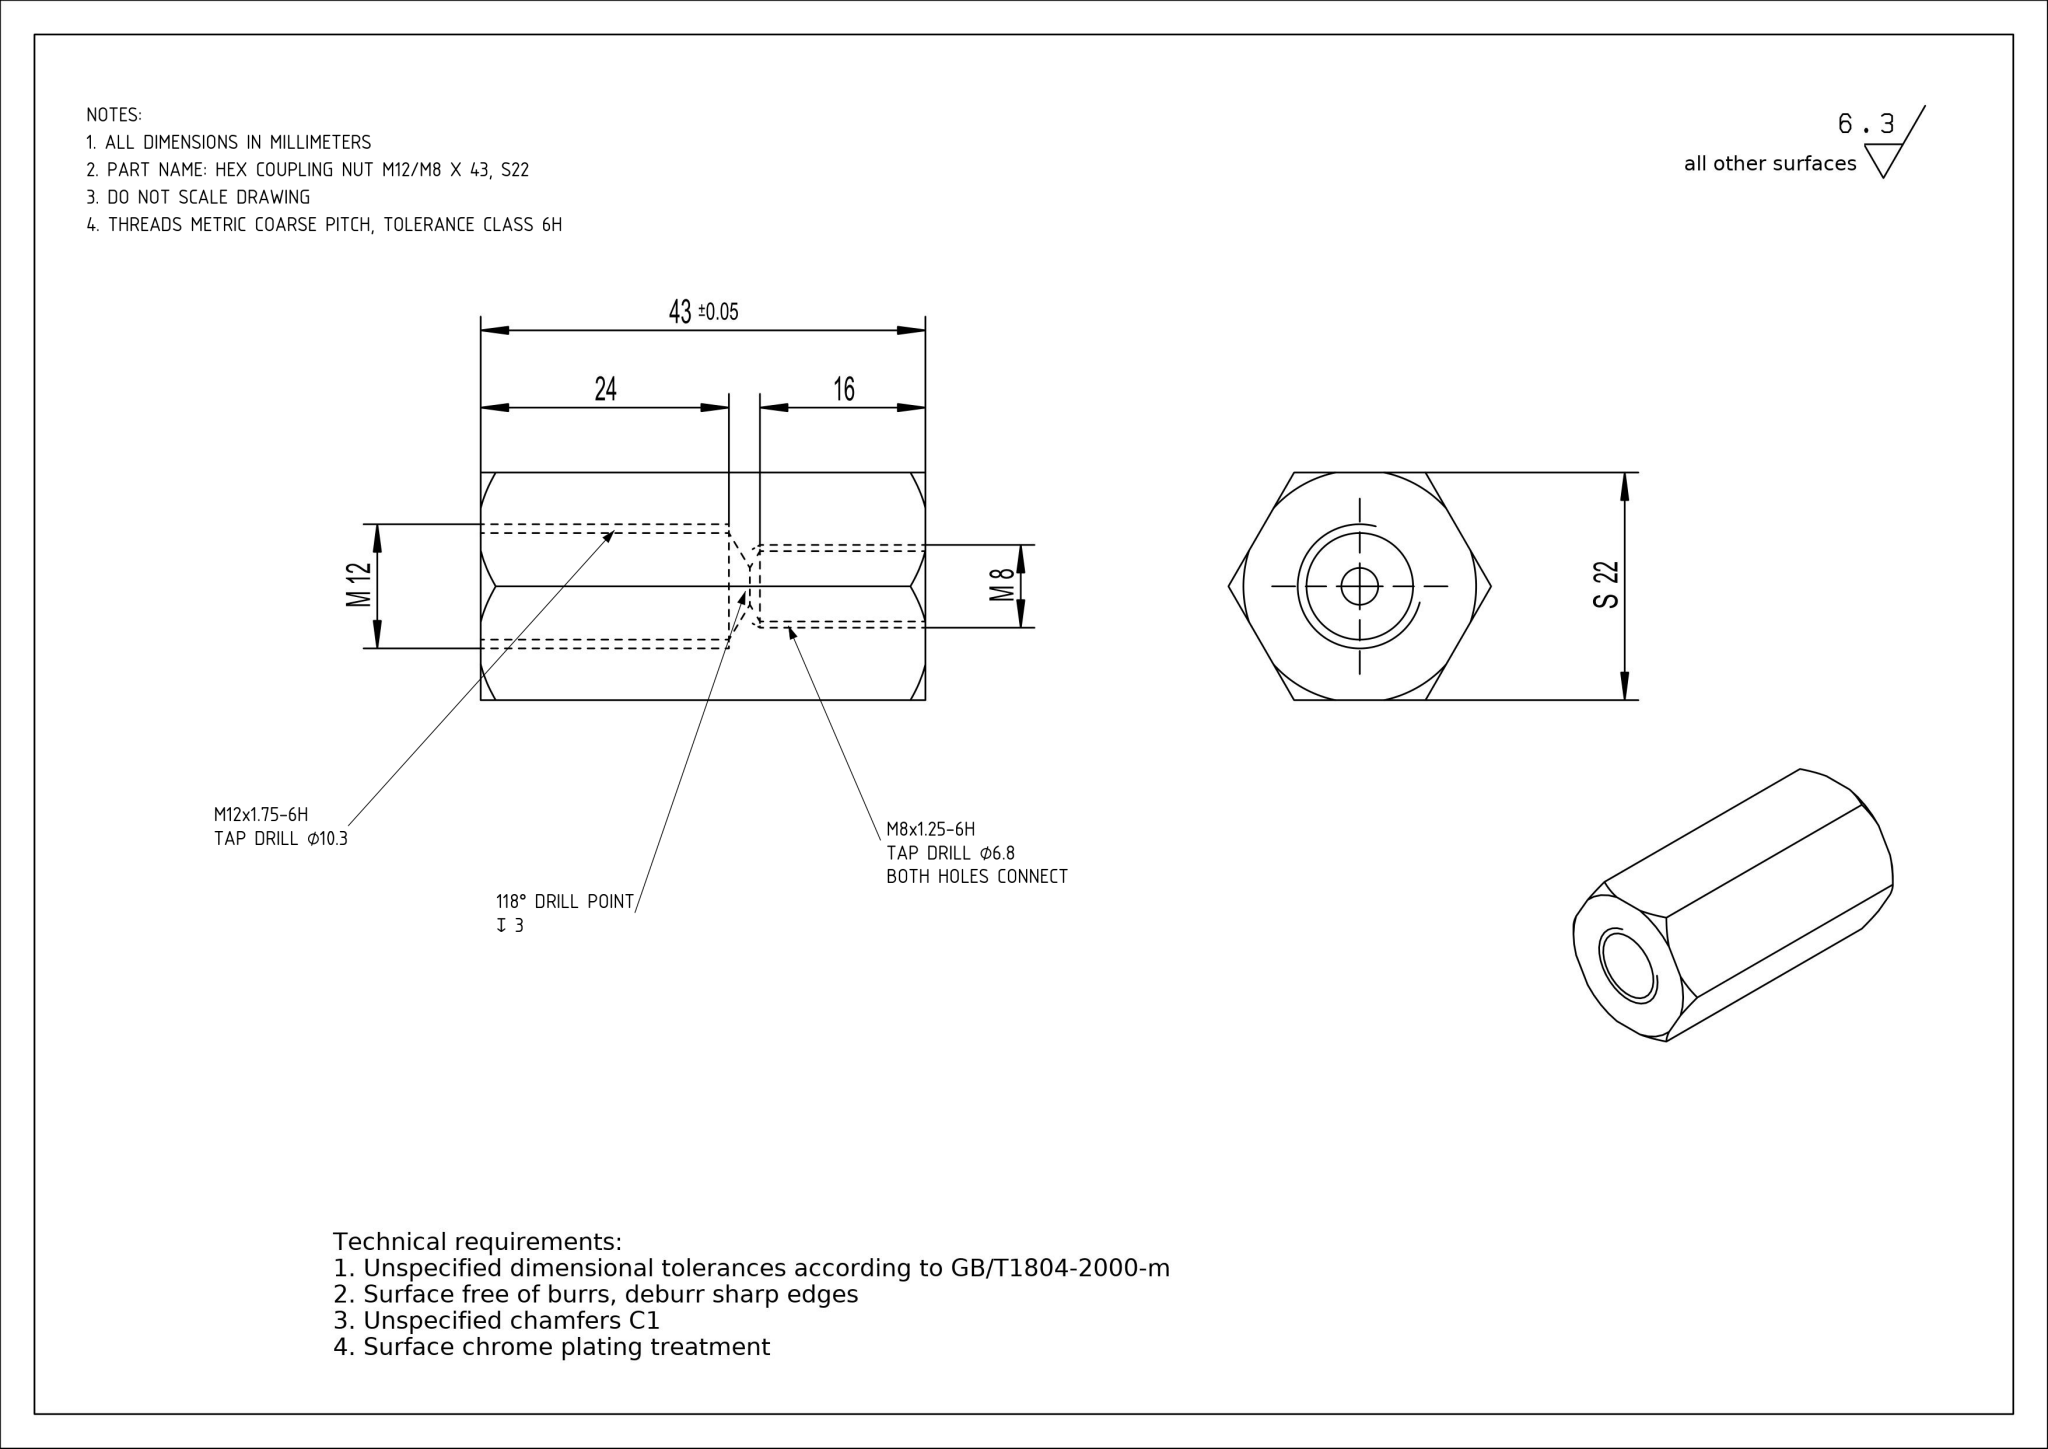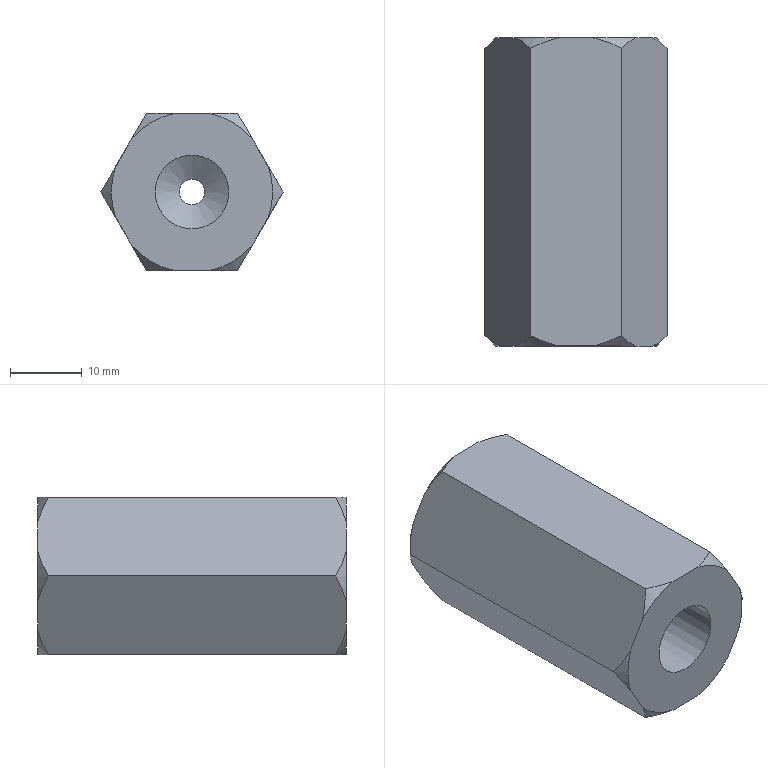Part | NX | mm | 1 solid | 24 faces | box 25.4 x 43 x 22 mm | volume 15315 mm3 | cone 14 | plane 8 | cylinder 2 | commonest cylinder face diameters 6.8 x1 10.3 x1
STEP:
#1=CARTESIAN_POINT('',(0.,0.,0.));
#2=DIRECTION('',(0.,0.,1.));
#3=DIRECTION('',(1.,0.,0.));
#4=AXIS2_PLACEMENT_3D('',#1,#2,#3);
#5=(LENGTH_UNIT()NAMED_UNIT(*)SI_UNIT(.MILLI.,.METRE.));
#6=UNCERTAINTY_MEASURE_WITH_UNIT(LENGTH_MEASURE(0.0508),#5,'','');
#7=(NAMED_UNIT(*)PLANE_ANGLE_UNIT()SI_UNIT($,.RADIAN.));
#8=PLANE_ANGLE_MEASURE_WITH_UNIT(PLANE_ANGLE_MEASURE(0.01745),#7);
#9=DIMENSIONAL_EXPONENTS(0.,0.,0.,0.,0.,0.,0.);
#10=(CONVERSION_BASED_UNIT('',#8)NAMED_UNIT(#9)PLANE_ANGLE_UNIT());
#11=(NAMED_UNIT(*)SI_UNIT($,.STERADIAN.)SOLID_ANGLE_UNIT());
#12=(GEOMETRIC_REPRESENTATION_CONTEXT(3)GLOBAL_UNCERTAINTY_ASSIGNED_CONTEXT((#6))GLOBAL_UNIT_ASSIGNED_CONTEXT((#5,#10,#11))REPRESENTATION_CONTEXT('',''));
#13=SHAPE_REPRESENTATION('',(#4),#12);
#14=CARTESIAN_POINT('',(0.,0.,5.15));
#15=VERTEX_POINT('',#14);
#16=CARTESIAN_POINT('',(0.,0.,0.));
#17=DIRECTION('',(0.,1.,0.));
#18=DIRECTION('',(0.,0.,1.));
#19=AXIS2_PLACEMENT_3D('',#16,#17,#18);
#20=CIRCLE('',#19,5.15);
#21=EDGE_CURVE('',#15,#15,#20,.T.);
#22=ORIENTED_EDGE('',*,*,#21,.T.);
#23=EDGE_LOOP('',(#22));
#24=FACE_BOUND('',#23,.T.);
#25=CARTESIAN_POINT('',(-8.347,0.,7.543));
#26=VERTEX_POINT('',#25);
#27=CARTESIAN_POINT('',(-2.358,0.,11.));
#28=VERTEX_POINT('',#27);
#29=CARTESIAN_POINT('',(0.,0.,-0.));
#30=DIRECTION('',(0.,1.,0.));
#31=DIRECTION('',(-1.,0.,-0.));
#32=AXIS2_PLACEMENT_3D('',#29,#30,#31);
#33=CIRCLE('',#32,11.25);
#34=EDGE_CURVE('',#26,#28,#33,.T.);
#35=ORIENTED_EDGE('',*,*,#34,.F.);
#36=CARTESIAN_POINT('',(-10.706,0.,3.457));
#37=VERTEX_POINT('',#36);
#38=CARTESIAN_POINT('',(-6.351,0.,11.));
#39=DIRECTION('',(-0.5,0.,-0.866));
#40=VECTOR('',#39,1.);
#41=LINE('',#38,#40);
#42=EDGE_CURVE('',#26,#37,#41,.T.);
#43=ORIENTED_EDGE('',*,*,#42,.T.);
#44=CARTESIAN_POINT('',(-10.706,0.,-3.457));
#45=VERTEX_POINT('',#44);
#46=CARTESIAN_POINT('',(0.,0.,-0.));
#47=DIRECTION('',(0.,1.,0.));
#48=DIRECTION('',(-1.,0.,-0.));
#49=AXIS2_PLACEMENT_3D('',#46,#47,#48);
#50=CIRCLE('',#49,11.25);
#51=EDGE_CURVE('',#45,#37,#50,.T.);
#52=ORIENTED_EDGE('',*,*,#51,.F.);
#53=CARTESIAN_POINT('',(-8.347,0.,-7.543));
#54=VERTEX_POINT('',#53);
#55=CARTESIAN_POINT('',(-12.702,0.,0.));
#56=DIRECTION('',(0.5,0.,-0.866));
#57=VECTOR('',#56,1.);
#58=LINE('',#55,#57);
#59=EDGE_CURVE('',#45,#54,#58,.T.);
#60=ORIENTED_EDGE('',*,*,#59,.T.);
#61=CARTESIAN_POINT('',(-2.358,0.,-11.));
#62=VERTEX_POINT('',#61);
#63=CARTESIAN_POINT('',(0.,0.,-0.));
#64=DIRECTION('',(0.,1.,0.));
#65=DIRECTION('',(-1.,0.,-0.));
#66=AXIS2_PLACEMENT_3D('',#63,#64,#65);
#67=CIRCLE('',#66,11.25);
#68=EDGE_CURVE('',#62,#54,#67,.T.);
#69=ORIENTED_EDGE('',*,*,#68,.F.);
#70=CARTESIAN_POINT('',(2.358,0.,-11.));
#71=VERTEX_POINT('',#70);
#72=CARTESIAN_POINT('',(-6.351,0.,-11.));
#73=DIRECTION('',(1.,0.,-0.));
#74=VECTOR('',#73,1.);
#75=LINE('',#72,#74);
#76=EDGE_CURVE('',#62,#71,#75,.T.);
#77=ORIENTED_EDGE('',*,*,#76,.T.);
#78=CARTESIAN_POINT('',(8.347,0.,-7.543));
#79=VERTEX_POINT('',#78);
#80=CARTESIAN_POINT('',(0.,0.,-0.));
#81=DIRECTION('',(0.,1.,0.));
#82=DIRECTION('',(-1.,0.,-0.));
#83=AXIS2_PLACEMENT_3D('',#80,#81,#82);
#84=CIRCLE('',#83,11.25);
#85=EDGE_CURVE('',#79,#71,#84,.T.);
#86=ORIENTED_EDGE('',*,*,#85,.F.);
#87=CARTESIAN_POINT('',(10.706,0.,-3.457));
#88=VERTEX_POINT('',#87);
#89=CARTESIAN_POINT('',(6.351,0.,-11.));
#90=DIRECTION('',(0.5,0.,0.866));
#91=VECTOR('',#90,1.);
#92=LINE('',#89,#91);
#93=EDGE_CURVE('',#79,#88,#92,.T.);
#94=ORIENTED_EDGE('',*,*,#93,.T.);
#95=CARTESIAN_POINT('',(10.706,0.,3.457));
#96=VERTEX_POINT('',#95);
#97=CARTESIAN_POINT('',(0.,0.,-0.));
#98=DIRECTION('',(0.,1.,0.));
#99=DIRECTION('',(-1.,0.,-0.));
#100=AXIS2_PLACEMENT_3D('',#97,#98,#99);
#101=CIRCLE('',#100,11.25);
#102=EDGE_CURVE('',#96,#88,#101,.T.);
#103=ORIENTED_EDGE('',*,*,#102,.F.);
#104=CARTESIAN_POINT('',(8.347,0.,7.543));
#105=VERTEX_POINT('',#104);
#106=CARTESIAN_POINT('',(12.702,0.,-0.));
#107=DIRECTION('',(-0.5,0.,0.866));
#108=VECTOR('',#107,1.);
#109=LINE('',#106,#108);
#110=EDGE_CURVE('',#96,#105,#109,.T.);
#111=ORIENTED_EDGE('',*,*,#110,.T.);
#112=CARTESIAN_POINT('',(2.358,0.,11.));
#113=VERTEX_POINT('',#112);
#114=CARTESIAN_POINT('',(0.,0.,-0.));
#115=DIRECTION('',(0.,1.,0.));
#116=DIRECTION('',(-1.,0.,-0.));
#117=AXIS2_PLACEMENT_3D('',#114,#115,#116);
#118=CIRCLE('',#117,11.25);
#119=EDGE_CURVE('',#113,#105,#118,.T.);
#120=ORIENTED_EDGE('',*,*,#119,.F.);
#121=CARTESIAN_POINT('',(6.351,0.,11.));
#122=DIRECTION('',(-1.,0.,0.));
#123=VECTOR('',#122,1.);
#124=LINE('',#121,#123);
#125=EDGE_CURVE('',#113,#28,#124,.T.);
#126=ORIENTED_EDGE('',*,*,#125,.T.);
#127=EDGE_LOOP('',(#35,#43,#52,#60,#69,#77,#86,#94,#103,#111,#120,#126));
#128=FACE_BOUND('',#127,.T.);
#129=CARTESIAN_POINT('',(0.,0.,0.));
#130=DIRECTION('',(0.,-1.,0.));
#131=DIRECTION('',(0.,0.,-1.));
#132=AXIS2_PLACEMENT_3D('',#129,#130,#131);
#133=PLANE('',#132);
#134=ADVANCED_FACE('',(#24,#128),#133,.T.);
#135=CARTESIAN_POINT('',(-6.351,1.452,-11.));
#136=VERTEX_POINT('',#135);
#137=CARTESIAN_POINT('',(-6.351,41.548,-11.));
#138=VERTEX_POINT('',#137);
#139=CARTESIAN_POINT('',(-6.351,0.,-11.));
#140=DIRECTION('',(0.,1.,0.));
#141=VECTOR('',#140,1.);
#142=LINE('',#139,#141);
#143=EDGE_CURVE('',#136,#138,#142,.T.);
#144=ORIENTED_EDGE('',*,*,#143,.F.);
#145=CARTESIAN_POINT('',(-6.351,1.452,-11.));
#146=CARTESIAN_POINT('',(-6.985,0.8177,-9.902));
#147=CARTESIAN_POINT('',(-7.653,0.2911,-8.745));
#148=CARTESIAN_POINT('',(-8.347,-0.,-7.543));
#149=B_SPLINE_CURVE_WITH_KNOTS('',3,(#145,#146,#147,#148),.UNSPECIFIED.,.F.,.F.,(4,4),(0.,1.),.UNSPECIFIED.);
#150=EDGE_CURVE('',#136,#54,#149,.T.);
#151=ORIENTED_EDGE('',*,*,#150,.T.);
#152=ORIENTED_EDGE('',*,*,#59,.F.);
#153=CARTESIAN_POINT('',(-12.702,1.452,0.));
#154=VERTEX_POINT('',#153);
#155=CARTESIAN_POINT('',(-10.706,-0.,-3.457));
#156=CARTESIAN_POINT('',(-11.399,0.2907,-2.257));
#157=CARTESIAN_POINT('',(-12.071,0.8206,-1.093));
#158=CARTESIAN_POINT('',(-12.702,1.452,0.));
#159=B_SPLINE_CURVE_WITH_KNOTS('',3,(#155,#156,#157,#158),.UNSPECIFIED.,.F.,.F.,(4,4),(0.,1.),.UNSPECIFIED.);
#160=EDGE_CURVE('',#45,#154,#159,.T.);
#161=ORIENTED_EDGE('',*,*,#160,.T.);
#162=CARTESIAN_POINT('',(-12.702,41.548,0.));
#163=VERTEX_POINT('',#162);
#164=CARTESIAN_POINT('',(-12.702,0.,0.));
#165=DIRECTION('',(0.,1.,0.));
#166=VECTOR('',#165,1.);
#167=LINE('',#164,#166);
#168=EDGE_CURVE('',#154,#163,#167,.T.);
#169=ORIENTED_EDGE('',*,*,#168,.T.);
#170=CARTESIAN_POINT('',(-10.706,43.,-3.457));
#171=VERTEX_POINT('',#170);
#172=CARTESIAN_POINT('',(-10.706,43.,-3.457));
#173=CARTESIAN_POINT('',(-11.399,42.709,-2.257));
#174=CARTESIAN_POINT('',(-12.071,42.179,-1.093));
#175=CARTESIAN_POINT('',(-12.702,41.548,0.));
#176=B_SPLINE_CURVE_WITH_KNOTS('',3,(#172,#173,#174,#175),.UNSPECIFIED.,.F.,.F.,(4,4),(0.,1.),.UNSPECIFIED.);
#177=EDGE_CURVE('',#171,#163,#176,.T.);
#178=ORIENTED_EDGE('',*,*,#177,.F.);
#179=CARTESIAN_POINT('',(-8.347,43.,-7.543));
#180=VERTEX_POINT('',#179);
#181=CARTESIAN_POINT('',(-12.702,43.,0.));
#182=DIRECTION('',(0.5,0.,-0.866));
#183=VECTOR('',#182,1.);
#184=LINE('',#181,#183);
#185=EDGE_CURVE('',#171,#180,#184,.T.);
#186=ORIENTED_EDGE('',*,*,#185,.T.);
#187=CARTESIAN_POINT('',(-6.351,41.548,-11.));
#188=CARTESIAN_POINT('',(-6.985,42.182,-9.902));
#189=CARTESIAN_POINT('',(-7.653,42.709,-8.745));
#190=CARTESIAN_POINT('',(-8.347,43.,-7.543));
#191=B_SPLINE_CURVE_WITH_KNOTS('',3,(#187,#188,#189,#190),.UNSPECIFIED.,.F.,.F.,(4,4),(0.,1.),.UNSPECIFIED.);
#192=EDGE_CURVE('',#138,#180,#191,.T.);
#193=ORIENTED_EDGE('',*,*,#192,.F.);
#194=EDGE_LOOP('',(#144,#151,#152,#161,#169,#178,#186,#193));
#195=FACE_OUTER_BOUND('',#194,.T.);
#196=CARTESIAN_POINT('',(-12.702,0.,0.));
#197=DIRECTION('',(0.866,0.,0.5));
#198=DIRECTION('',(0.5,0.,-0.866));
#199=AXIS2_PLACEMENT_3D('',#196,#197,#198);
#200=PLANE('',#199);
#201=ADVANCED_FACE('',(#195),#200,.F.);
#202=CARTESIAN_POINT('',(6.351,1.452,-11.));
#203=VERTEX_POINT('',#202);
#204=CARTESIAN_POINT('',(6.351,41.548,-11.));
#205=VERTEX_POINT('',#204);
#206=CARTESIAN_POINT('',(6.351,0.,-11.));
#207=DIRECTION('',(0.,1.,0.));
#208=VECTOR('',#207,1.);
#209=LINE('',#206,#208);
#210=EDGE_CURVE('',#203,#205,#209,.T.);
#211=ORIENTED_EDGE('',*,*,#210,.F.);
#212=CARTESIAN_POINT('',(6.351,1.452,-11.));
#213=CARTESIAN_POINT('',(5.077,0.8149,-11.));
#214=CARTESIAN_POINT('',(3.751,0.2919,-11.));
#215=CARTESIAN_POINT('',(2.358,-0.,-11.));
#216=B_SPLINE_CURVE_WITH_KNOTS('',3,(#212,#213,#214,#215),.UNSPECIFIED.,.F.,.F.,(4,4),(0.,1.),.UNSPECIFIED.);
#217=EDGE_CURVE('',#203,#71,#216,.T.);
#218=ORIENTED_EDGE('',*,*,#217,.T.);
#219=ORIENTED_EDGE('',*,*,#76,.F.);
#220=CARTESIAN_POINT('',(-2.358,-0.,-11.));
#221=CARTESIAN_POINT('',(-3.752,0.292,-11.));
#222=CARTESIAN_POINT('',(-5.085,0.8187,-11.));
#223=CARTESIAN_POINT('',(-6.351,1.452,-11.));
#224=B_SPLINE_CURVE_WITH_KNOTS('',3,(#220,#221,#222,#223),.UNSPECIFIED.,.F.,.F.,(4,4),(0.,1.),.UNSPECIFIED.);
#225=EDGE_CURVE('',#62,#136,#224,.T.);
#226=ORIENTED_EDGE('',*,*,#225,.T.);
#227=ORIENTED_EDGE('',*,*,#143,.T.);
#228=CARTESIAN_POINT('',(-2.358,43.,-11.));
#229=VERTEX_POINT('',#228);
#230=CARTESIAN_POINT('',(-2.358,43.,-11.));
#231=CARTESIAN_POINT('',(-3.752,42.708,-11.));
#232=CARTESIAN_POINT('',(-5.085,42.181,-11.));
#233=CARTESIAN_POINT('',(-6.351,41.548,-11.));
#234=B_SPLINE_CURVE_WITH_KNOTS('',3,(#230,#231,#232,#233),.UNSPECIFIED.,.F.,.F.,(4,4),(0.,1.),.UNSPECIFIED.);
#235=EDGE_CURVE('',#229,#138,#234,.T.);
#236=ORIENTED_EDGE('',*,*,#235,.F.);
#237=CARTESIAN_POINT('',(2.358,43.,-11.));
#238=VERTEX_POINT('',#237);
#239=CARTESIAN_POINT('',(-6.351,43.,-11.));
#240=DIRECTION('',(1.,0.,-0.));
#241=VECTOR('',#240,1.);
#242=LINE('',#239,#241);
#243=EDGE_CURVE('',#229,#238,#242,.T.);
#244=ORIENTED_EDGE('',*,*,#243,.T.);
#245=CARTESIAN_POINT('',(6.351,41.548,-11.));
#246=CARTESIAN_POINT('',(5.077,42.185,-11.));
#247=CARTESIAN_POINT('',(3.751,42.708,-11.));
#248=CARTESIAN_POINT('',(2.358,43.,-11.));
#249=B_SPLINE_CURVE_WITH_KNOTS('',3,(#245,#246,#247,#248),.UNSPECIFIED.,.F.,.F.,(4,4),(0.,1.),.UNSPECIFIED.);
#250=EDGE_CURVE('',#205,#238,#249,.T.);
#251=ORIENTED_EDGE('',*,*,#250,.F.);
#252=EDGE_LOOP('',(#211,#218,#219,#226,#227,#236,#244,#251));
#253=FACE_OUTER_BOUND('',#252,.T.);
#254=CARTESIAN_POINT('',(-6.351,0.,-11.));
#255=DIRECTION('',(0.,0.,1.));
#256=DIRECTION('',(1.,0.,-0.));
#257=AXIS2_PLACEMENT_3D('',#254,#255,#256);
#258=PLANE('',#257);
#259=ADVANCED_FACE('',(#253),#258,.F.);
#260=CARTESIAN_POINT('',(12.702,1.452,-0.));
#261=VERTEX_POINT('',#260);
#262=CARTESIAN_POINT('',(12.702,41.548,-0.));
#263=VERTEX_POINT('',#262);
#264=CARTESIAN_POINT('',(12.702,0.,-0.));
#265=DIRECTION('',(0.,1.,0.));
#266=VECTOR('',#265,1.);
#267=LINE('',#264,#266);
#268=EDGE_CURVE('',#261,#263,#267,.T.);
#269=ORIENTED_EDGE('',*,*,#268,.F.);
#270=CARTESIAN_POINT('',(12.702,1.452,-0.));
#271=CARTESIAN_POINT('',(12.068,0.8177,-1.098));
#272=CARTESIAN_POINT('',(11.4,0.2911,-2.255));
#273=CARTESIAN_POINT('',(10.706,0.,-3.457));
#274=B_SPLINE_CURVE_WITH_KNOTS('',3,(#270,#271,#272,#273),.UNSPECIFIED.,.F.,.F.,(4,4),(0.,1.),.UNSPECIFIED.);
#275=EDGE_CURVE('',#261,#88,#274,.T.);
#276=ORIENTED_EDGE('',*,*,#275,.T.);
#277=ORIENTED_EDGE('',*,*,#93,.F.);
#278=CARTESIAN_POINT('',(8.347,0.,-7.543));
#279=CARTESIAN_POINT('',(7.654,0.2907,-8.743));
#280=CARTESIAN_POINT('',(6.982,0.8206,-9.907));
#281=CARTESIAN_POINT('',(6.351,1.452,-11.));
#282=B_SPLINE_CURVE_WITH_KNOTS('',3,(#278,#279,#280,#281),.UNSPECIFIED.,.F.,.F.,(4,4),(0.,1.),.UNSPECIFIED.);
#283=EDGE_CURVE('',#79,#203,#282,.T.);
#284=ORIENTED_EDGE('',*,*,#283,.T.);
#285=ORIENTED_EDGE('',*,*,#210,.T.);
#286=CARTESIAN_POINT('',(8.347,43.,-7.543));
#287=VERTEX_POINT('',#286);
#288=CARTESIAN_POINT('',(8.347,43.,-7.543));
#289=CARTESIAN_POINT('',(7.654,42.709,-8.743));
#290=CARTESIAN_POINT('',(6.982,42.179,-9.907));
#291=CARTESIAN_POINT('',(6.351,41.548,-11.));
#292=B_SPLINE_CURVE_WITH_KNOTS('',3,(#288,#289,#290,#291),.UNSPECIFIED.,.F.,.F.,(4,4),(0.,1.),.UNSPECIFIED.);
#293=EDGE_CURVE('',#287,#205,#292,.T.);
#294=ORIENTED_EDGE('',*,*,#293,.F.);
#295=CARTESIAN_POINT('',(10.706,43.,-3.457));
#296=VERTEX_POINT('',#295);
#297=CARTESIAN_POINT('',(6.351,43.,-11.));
#298=DIRECTION('',(0.5,0.,0.866));
#299=VECTOR('',#298,1.);
#300=LINE('',#297,#299);
#301=EDGE_CURVE('',#287,#296,#300,.T.);
#302=ORIENTED_EDGE('',*,*,#301,.T.);
#303=CARTESIAN_POINT('',(12.702,41.548,-0.));
#304=CARTESIAN_POINT('',(12.068,42.182,-1.098));
#305=CARTESIAN_POINT('',(11.4,42.709,-2.255));
#306=CARTESIAN_POINT('',(10.706,43.,-3.457));
#307=B_SPLINE_CURVE_WITH_KNOTS('',3,(#303,#304,#305,#306),.UNSPECIFIED.,.F.,.F.,(4,4),(0.,1.),.UNSPECIFIED.);
#308=EDGE_CURVE('',#263,#296,#307,.T.);
#309=ORIENTED_EDGE('',*,*,#308,.F.);
#310=EDGE_LOOP('',(#269,#276,#277,#284,#285,#294,#302,#309));
#311=FACE_OUTER_BOUND('',#310,.T.);
#312=CARTESIAN_POINT('',(6.351,0.,-11.));
#313=DIRECTION('',(-0.866,0.,0.5));
#314=DIRECTION('',(0.5,0.,0.866));
#315=AXIS2_PLACEMENT_3D('',#312,#313,#314);
#316=PLANE('',#315);
#317=ADVANCED_FACE('',(#311),#316,.F.);
#318=CARTESIAN_POINT('',(6.351,1.452,11.));
#319=VERTEX_POINT('',#318);
#320=CARTESIAN_POINT('',(6.351,41.548,11.));
#321=VERTEX_POINT('',#320);
#322=CARTESIAN_POINT('',(6.351,0.,11.));
#323=DIRECTION('',(0.,1.,0.));
#324=VECTOR('',#323,1.);
#325=LINE('',#322,#324);
#326=EDGE_CURVE('',#319,#321,#325,.T.);
#327=ORIENTED_EDGE('',*,*,#326,.F.);
#328=CARTESIAN_POINT('',(6.351,1.452,11.));
#329=CARTESIAN_POINT('',(6.985,0.8177,9.902));
#330=CARTESIAN_POINT('',(7.653,0.2911,8.745));
#331=CARTESIAN_POINT('',(8.347,-0.,7.543));
#332=B_SPLINE_CURVE_WITH_KNOTS('',3,(#328,#329,#330,#331),.UNSPECIFIED.,.F.,.F.,(4,4),(0.,1.),.UNSPECIFIED.);
#333=EDGE_CURVE('',#319,#105,#332,.T.);
#334=ORIENTED_EDGE('',*,*,#333,.T.);
#335=ORIENTED_EDGE('',*,*,#110,.F.);
#336=CARTESIAN_POINT('',(10.706,-0.,3.457));
#337=CARTESIAN_POINT('',(11.399,0.2907,2.257));
#338=CARTESIAN_POINT('',(12.071,0.8206,1.093));
#339=CARTESIAN_POINT('',(12.702,1.452,-0.));
#340=B_SPLINE_CURVE_WITH_KNOTS('',3,(#336,#337,#338,#339),.UNSPECIFIED.,.F.,.F.,(4,4),(0.,1.),.UNSPECIFIED.);
#341=EDGE_CURVE('',#96,#261,#340,.T.);
#342=ORIENTED_EDGE('',*,*,#341,.T.);
#343=ORIENTED_EDGE('',*,*,#268,.T.);
#344=CARTESIAN_POINT('',(10.706,43.,3.457));
#345=VERTEX_POINT('',#344);
#346=CARTESIAN_POINT('',(10.706,43.,3.457));
#347=CARTESIAN_POINT('',(11.399,42.709,2.257));
#348=CARTESIAN_POINT('',(12.071,42.179,1.093));
#349=CARTESIAN_POINT('',(12.702,41.548,-0.));
#350=B_SPLINE_CURVE_WITH_KNOTS('',3,(#346,#347,#348,#349),.UNSPECIFIED.,.F.,.F.,(4,4),(0.,1.),.UNSPECIFIED.);
#351=EDGE_CURVE('',#345,#263,#350,.T.);
#352=ORIENTED_EDGE('',*,*,#351,.F.);
#353=CARTESIAN_POINT('',(8.347,43.,7.543));
#354=VERTEX_POINT('',#353);
#355=CARTESIAN_POINT('',(12.702,43.,-0.));
#356=DIRECTION('',(-0.5,0.,0.866));
#357=VECTOR('',#356,1.);
#358=LINE('',#355,#357);
#359=EDGE_CURVE('',#345,#354,#358,.T.);
#360=ORIENTED_EDGE('',*,*,#359,.T.);
#361=CARTESIAN_POINT('',(6.351,41.548,11.));
#362=CARTESIAN_POINT('',(6.985,42.182,9.902));
#363=CARTESIAN_POINT('',(7.653,42.709,8.745));
#364=CARTESIAN_POINT('',(8.347,43.,7.543));
#365=B_SPLINE_CURVE_WITH_KNOTS('',3,(#361,#362,#363,#364),.UNSPECIFIED.,.F.,.F.,(4,4),(0.,1.),.UNSPECIFIED.);
#366=EDGE_CURVE('',#321,#354,#365,.T.);
#367=ORIENTED_EDGE('',*,*,#366,.F.);
#368=EDGE_LOOP('',(#327,#334,#335,#342,#343,#352,#360,#367));
#369=FACE_OUTER_BOUND('',#368,.T.);
#370=CARTESIAN_POINT('',(12.702,0.,-0.));
#371=DIRECTION('',(-0.866,0.,-0.5));
#372=DIRECTION('',(-0.5,0.,0.866));
#373=AXIS2_PLACEMENT_3D('',#370,#371,#372);
#374=PLANE('',#373);
#375=ADVANCED_FACE('',(#369),#374,.F.);
#376=CARTESIAN_POINT('',(-6.351,1.452,11.));
#377=VERTEX_POINT('',#376);
#378=CARTESIAN_POINT('',(-6.351,41.548,11.));
#379=VERTEX_POINT('',#378);
#380=CARTESIAN_POINT('',(-6.351,0.,11.));
#381=DIRECTION('',(0.,1.,0.));
#382=VECTOR('',#381,1.);
#383=LINE('',#380,#382);
#384=EDGE_CURVE('',#377,#379,#383,.T.);
#385=ORIENTED_EDGE('',*,*,#384,.F.);
#386=CARTESIAN_POINT('',(-6.351,1.452,11.));
#387=CARTESIAN_POINT('',(-5.077,0.8149,11.));
#388=CARTESIAN_POINT('',(-3.751,0.2919,11.));
#389=CARTESIAN_POINT('',(-2.358,-0.,11.));
#390=B_SPLINE_CURVE_WITH_KNOTS('',3,(#386,#387,#388,#389),.UNSPECIFIED.,.F.,.F.,(4,4),(0.,1.),.UNSPECIFIED.);
#391=EDGE_CURVE('',#377,#28,#390,.T.);
#392=ORIENTED_EDGE('',*,*,#391,.T.);
#393=ORIENTED_EDGE('',*,*,#125,.F.);
#394=CARTESIAN_POINT('',(2.358,-0.,11.));
#395=CARTESIAN_POINT('',(3.752,0.292,11.));
#396=CARTESIAN_POINT('',(5.085,0.8187,11.));
#397=CARTESIAN_POINT('',(6.351,1.452,11.));
#398=B_SPLINE_CURVE_WITH_KNOTS('',3,(#394,#395,#396,#397),.UNSPECIFIED.,.F.,.F.,(4,4),(0.,1.),.UNSPECIFIED.);
#399=EDGE_CURVE('',#113,#319,#398,.T.);
#400=ORIENTED_EDGE('',*,*,#399,.T.);
#401=ORIENTED_EDGE('',*,*,#326,.T.);
#402=CARTESIAN_POINT('',(2.358,43.,11.));
#403=VERTEX_POINT('',#402);
#404=CARTESIAN_POINT('',(2.358,43.,11.));
#405=CARTESIAN_POINT('',(3.752,42.708,11.));
#406=CARTESIAN_POINT('',(5.085,42.181,11.));
#407=CARTESIAN_POINT('',(6.351,41.548,11.));
#408=B_SPLINE_CURVE_WITH_KNOTS('',3,(#404,#405,#406,#407),.UNSPECIFIED.,.F.,.F.,(4,4),(0.,1.),.UNSPECIFIED.);
#409=EDGE_CURVE('',#403,#321,#408,.T.);
#410=ORIENTED_EDGE('',*,*,#409,.F.);
#411=CARTESIAN_POINT('',(-2.358,43.,11.));
#412=VERTEX_POINT('',#411);
#413=CARTESIAN_POINT('',(6.351,43.,11.));
#414=DIRECTION('',(-1.,0.,0.));
#415=VECTOR('',#414,1.);
#416=LINE('',#413,#415);
#417=EDGE_CURVE('',#403,#412,#416,.T.);
#418=ORIENTED_EDGE('',*,*,#417,.T.);
#419=CARTESIAN_POINT('',(-6.351,41.548,11.));
#420=CARTESIAN_POINT('',(-5.077,42.185,11.));
#421=CARTESIAN_POINT('',(-3.751,42.708,11.));
#422=CARTESIAN_POINT('',(-2.358,43.,11.));
#423=B_SPLINE_CURVE_WITH_KNOTS('',3,(#419,#420,#421,#422),.UNSPECIFIED.,.F.,.F.,(4,4),(0.,1.),.UNSPECIFIED.);
#424=EDGE_CURVE('',#379,#412,#423,.T.);
#425=ORIENTED_EDGE('',*,*,#424,.F.);
#426=EDGE_LOOP('',(#385,#392,#393,#400,#401,#410,#418,#425));
#427=FACE_OUTER_BOUND('',#426,.T.);
#428=CARTESIAN_POINT('',(6.351,0.,11.));
#429=DIRECTION('',(-0.,0.,-1.));
#430=DIRECTION('',(-1.,0.,0.));
#431=AXIS2_PLACEMENT_3D('',#428,#429,#430);
#432=PLANE('',#431);
#433=ADVANCED_FACE('',(#427),#432,.F.);
#434=ORIENTED_EDGE('',*,*,#168,.F.);
#435=CARTESIAN_POINT('',(-12.702,1.452,0.));
#436=CARTESIAN_POINT('',(-12.068,0.8177,1.098));
#437=CARTESIAN_POINT('',(-11.4,0.2911,2.255));
#438=CARTESIAN_POINT('',(-10.706,0.,3.457));
#439=B_SPLINE_CURVE_WITH_KNOTS('',3,(#435,#436,#437,#438),.UNSPECIFIED.,.F.,.F.,(4,4),(0.,1.),.UNSPECIFIED.);
#440=EDGE_CURVE('',#154,#37,#439,.T.);
#441=ORIENTED_EDGE('',*,*,#440,.T.);
#442=ORIENTED_EDGE('',*,*,#42,.F.);
#443=CARTESIAN_POINT('',(-8.347,0.,7.543));
#444=CARTESIAN_POINT('',(-7.654,0.2907,8.743));
#445=CARTESIAN_POINT('',(-6.982,0.8206,9.907));
#446=CARTESIAN_POINT('',(-6.351,1.452,11.));
#447=B_SPLINE_CURVE_WITH_KNOTS('',3,(#443,#444,#445,#446),.UNSPECIFIED.,.F.,.F.,(4,4),(0.,1.),.UNSPECIFIED.);
#448=EDGE_CURVE('',#26,#377,#447,.T.);
#449=ORIENTED_EDGE('',*,*,#448,.T.);
#450=ORIENTED_EDGE('',*,*,#384,.T.);
#451=CARTESIAN_POINT('',(-8.347,43.,7.543));
#452=VERTEX_POINT('',#451);
#453=CARTESIAN_POINT('',(-8.347,43.,7.543));
#454=CARTESIAN_POINT('',(-7.654,42.709,8.743));
#455=CARTESIAN_POINT('',(-6.982,42.179,9.907));
#456=CARTESIAN_POINT('',(-6.351,41.548,11.));
#457=B_SPLINE_CURVE_WITH_KNOTS('',3,(#453,#454,#455,#456),.UNSPECIFIED.,.F.,.F.,(4,4),(0.,1.),.UNSPECIFIED.);
#458=EDGE_CURVE('',#452,#379,#457,.T.);
#459=ORIENTED_EDGE('',*,*,#458,.F.);
#460=CARTESIAN_POINT('',(-10.706,43.,3.457));
#461=VERTEX_POINT('',#460);
#462=CARTESIAN_POINT('',(-6.351,43.,11.));
#463=DIRECTION('',(-0.5,0.,-0.866));
#464=VECTOR('',#463,1.);
#465=LINE('',#462,#464);
#466=EDGE_CURVE('',#452,#461,#465,.T.);
#467=ORIENTED_EDGE('',*,*,#466,.T.);
#468=CARTESIAN_POINT('',(-12.702,41.548,0.));
#469=CARTESIAN_POINT('',(-12.068,42.182,1.098));
#470=CARTESIAN_POINT('',(-11.4,42.709,2.255));
#471=CARTESIAN_POINT('',(-10.706,43.,3.457));
#472=B_SPLINE_CURVE_WITH_KNOTS('',3,(#468,#469,#470,#471),.UNSPECIFIED.,.F.,.F.,(4,4),(0.,1.),.UNSPECIFIED.);
#473=EDGE_CURVE('',#163,#461,#472,.T.);
#474=ORIENTED_EDGE('',*,*,#473,.F.);
#475=EDGE_LOOP('',(#434,#441,#442,#449,#450,#459,#467,#474));
#476=FACE_OUTER_BOUND('',#475,.T.);
#477=CARTESIAN_POINT('',(-6.351,0.,11.));
#478=DIRECTION('',(0.866,0.,-0.5));
#479=DIRECTION('',(-0.5,0.,-0.866));
#480=AXIS2_PLACEMENT_3D('',#477,#478,#479);
#481=PLANE('',#480);
#482=ADVANCED_FACE('',(#476),#481,.F.);
#483=CARTESIAN_POINT('',(0.,43.,-3.4));
#484=VERTEX_POINT('',#483);
#485=CARTESIAN_POINT('',(0.,43.,0.));
#486=DIRECTION('',(0.,-1.,0.));
#487=DIRECTION('',(0.,0.,-1.));
#488=AXIS2_PLACEMENT_3D('',#485,#486,#487);
#489=CIRCLE('',#488,3.4);
#490=EDGE_CURVE('',#484,#484,#489,.T.);
#491=ORIENTED_EDGE('',*,*,#490,.T.);
#492=EDGE_LOOP('',(#491));
#493=FACE_BOUND('',#492,.T.);
#494=ORIENTED_EDGE('',*,*,#466,.F.);
#495=CARTESIAN_POINT('',(0.,43.,0.));
#496=DIRECTION('',(0.,1.,0.));
#497=DIRECTION('',(-1.,0.,-0.));
#498=AXIS2_PLACEMENT_3D('',#495,#496,#497);
#499=CIRCLE('',#498,11.25);
#500=EDGE_CURVE('',#452,#412,#499,.T.);
#501=ORIENTED_EDGE('',*,*,#500,.T.);
#502=ORIENTED_EDGE('',*,*,#417,.F.);
#503=CARTESIAN_POINT('',(0.,43.,0.));
#504=DIRECTION('',(0.,1.,0.));
#505=DIRECTION('',(-1.,0.,-0.));
#506=AXIS2_PLACEMENT_3D('',#503,#504,#505);
#507=CIRCLE('',#506,11.25);
#508=EDGE_CURVE('',#403,#354,#507,.T.);
#509=ORIENTED_EDGE('',*,*,#508,.T.);
#510=ORIENTED_EDGE('',*,*,#359,.F.);
#511=CARTESIAN_POINT('',(0.,43.,0.));
#512=DIRECTION('',(0.,1.,0.));
#513=DIRECTION('',(-1.,0.,-0.));
#514=AXIS2_PLACEMENT_3D('',#511,#512,#513);
#515=CIRCLE('',#514,11.25);
#516=EDGE_CURVE('',#345,#296,#515,.T.);
#517=ORIENTED_EDGE('',*,*,#516,.T.);
#518=ORIENTED_EDGE('',*,*,#301,.F.);
#519=CARTESIAN_POINT('',(0.,43.,0.));
#520=DIRECTION('',(0.,1.,0.));
#521=DIRECTION('',(-1.,0.,-0.));
#522=AXIS2_PLACEMENT_3D('',#519,#520,#521);
#523=CIRCLE('',#522,11.25);
#524=EDGE_CURVE('',#287,#238,#523,.T.);
#525=ORIENTED_EDGE('',*,*,#524,.T.);
#526=ORIENTED_EDGE('',*,*,#243,.F.);
#527=CARTESIAN_POINT('',(0.,43.,0.));
#528=DIRECTION('',(0.,1.,0.));
#529=DIRECTION('',(-1.,0.,-0.));
#530=AXIS2_PLACEMENT_3D('',#527,#528,#529);
#531=CIRCLE('',#530,11.25);
#532=EDGE_CURVE('',#229,#180,#531,.T.);
#533=ORIENTED_EDGE('',*,*,#532,.T.);
#534=ORIENTED_EDGE('',*,*,#185,.F.);
#535=CARTESIAN_POINT('',(0.,43.,0.));
#536=DIRECTION('',(0.,1.,0.));
#537=DIRECTION('',(-1.,0.,-0.));
#538=AXIS2_PLACEMENT_3D('',#535,#536,#537);
#539=CIRCLE('',#538,11.25);
#540=EDGE_CURVE('',#171,#461,#539,.T.);
#541=ORIENTED_EDGE('',*,*,#540,.T.);
#542=EDGE_LOOP('',(#494,#501,#502,#509,#510,#517,#518,#525,#526,#533,#534,#541));
#543=FACE_BOUND('',#542,.T.);
#544=CARTESIAN_POINT('',(0.,43.,0.));
#545=DIRECTION('',(0.,-1.,0.));
#546=DIRECTION('',(0.,0.,-1.));
#547=AXIS2_PLACEMENT_3D('',#544,#545,#546);
#548=PLANE('',#547);
#549=ADVANCED_FACE('',(#493,#543),#548,.F.);
#550=CARTESIAN_POINT('',(0.,26.026,-1.779));
#551=VERTEX_POINT('',#550);
#552=CARTESIAN_POINT('',(0.,26.026,0.));
#553=DIRECTION('',(0.,-1.,0.));
#554=DIRECTION('',(0.,0.,-1.));
#555=AXIS2_PLACEMENT_3D('',#552,#553,#554);
#556=CIRCLE('',#555,1.779);
#557=EDGE_CURVE('',#551,#551,#556,.T.);
#558=ORIENTED_EDGE('',*,*,#557,.T.);
#559=EDGE_LOOP('',(#558));
#560=FACE_BOUND('',#559,.T.);
#561=CARTESIAN_POINT('',(0.,27.,-3.4));
#562=VERTEX_POINT('',#561);
#563=CARTESIAN_POINT('',(0.,27.,0.));
#564=DIRECTION('',(0.,1.,0.));
#565=DIRECTION('',(0.,0.,-1.));
#566=AXIS2_PLACEMENT_3D('',#563,#564,#565);
#567=CIRCLE('',#566,3.4);
#568=EDGE_CURVE('',#562,#562,#567,.T.);
#569=ORIENTED_EDGE('',*,*,#568,.T.);
#570=EDGE_LOOP('',(#569));
#571=FACE_BOUND('',#570,.T.);
#572=CARTESIAN_POINT('',(0.,27.,0.));
#573=DIRECTION('',(0.,1.,0.));
#574=DIRECTION('',(0.,-0.,1.));
#575=AXIS2_PLACEMENT_3D('',#572,#573,#574);
#576=CONICAL_SURFACE('',#575,3.4,59.);
#577=ADVANCED_FACE('',(#560,#571),#576,.F.);
#578=ORIENTED_EDGE('',*,*,#568,.F.);
#579=EDGE_LOOP('',(#578));
#580=FACE_BOUND('',#579,.T.);
#581=ORIENTED_EDGE('',*,*,#490,.F.);
#582=EDGE_LOOP('',(#581));
#583=FACE_BOUND('',#582,.T.);
#584=CARTESIAN_POINT('',(0.,43.,0.));
#585=DIRECTION('',(0.,-1.,0.));
#586=DIRECTION('',(0.,0.,-1.));
#587=AXIS2_PLACEMENT_3D('',#584,#585,#586);
#588=CYLINDRICAL_SURFACE('',#587,3.4);
#589=ADVANCED_FACE('',(#580,#583),#588,.F.);
#590=CARTESIAN_POINT('',(0.,24.,5.15));
#591=VERTEX_POINT('',#590);
#592=CARTESIAN_POINT('',(0.,24.,0.));
#593=DIRECTION('',(0.,-1.,0.));
#594=DIRECTION('',(0.,0.,1.));
#595=AXIS2_PLACEMENT_3D('',#592,#593,#594);
#596=CIRCLE('',#595,5.15);
#597=EDGE_CURVE('',#591,#591,#596,.T.);
#598=ORIENTED_EDGE('',*,*,#597,.T.);
#599=EDGE_LOOP('',(#598));
#600=FACE_BOUND('',#599,.T.);
#601=ORIENTED_EDGE('',*,*,#557,.F.);
#602=EDGE_LOOP('',(#601));
#603=FACE_BOUND('',#602,.T.);
#604=CARTESIAN_POINT('',(0.,24.,0.));
#605=DIRECTION('',(0.,-1.,0.));
#606=DIRECTION('',(0.,0.,-1.));
#607=AXIS2_PLACEMENT_3D('',#604,#605,#606);
#608=CONICAL_SURFACE('',#607,5.15,59.);
#609=ADVANCED_FACE('',(#600,#603),#608,.F.);
#610=ORIENTED_EDGE('',*,*,#597,.F.);
#611=EDGE_LOOP('',(#610));
#612=FACE_BOUND('',#611,.T.);
#613=ORIENTED_EDGE('',*,*,#21,.F.);
#614=EDGE_LOOP('',(#613));
#615=FACE_BOUND('',#614,.T.);
#616=CARTESIAN_POINT('',(0.,0.,0.));
#617=DIRECTION('',(0.,1.,0.));
#618=DIRECTION('',(0.,0.,1.));
#619=AXIS2_PLACEMENT_3D('',#616,#617,#618);
#620=CYLINDRICAL_SURFACE('',#619,5.15);
#621=ADVANCED_FACE('',(#612,#615),#620,.F.);
#622=ORIENTED_EDGE('',*,*,#424,.T.);
#623=ORIENTED_EDGE('',*,*,#500,.F.);
#624=ORIENTED_EDGE('',*,*,#458,.T.);
#625=EDGE_LOOP('',(#622,#623,#624));
#626=FACE_OUTER_BOUND('',#625,.T.);
#627=CARTESIAN_POINT('',(0.,43.,0.));
#628=DIRECTION('',(0.,-1.,0.));
#629=DIRECTION('',(0.,0.,1.));
#630=AXIS2_PLACEMENT_3D('',#627,#628,#629);
#631=CONICAL_SURFACE('',#630,11.25,45.);
#632=ADVANCED_FACE('',(#626),#631,.T.);
#633=ORIENTED_EDGE('',*,*,#177,.T.);
#634=ORIENTED_EDGE('',*,*,#473,.T.);
#635=ORIENTED_EDGE('',*,*,#540,.F.);
#636=EDGE_LOOP('',(#633,#634,#635));
#637=FACE_OUTER_BOUND('',#636,.T.);
#638=CARTESIAN_POINT('',(0.,43.,0.));
#639=DIRECTION('',(0.,-1.,0.));
#640=DIRECTION('',(0.,0.,1.));
#641=AXIS2_PLACEMENT_3D('',#638,#639,#640);
#642=CONICAL_SURFACE('',#641,11.25,45.);
#643=ADVANCED_FACE('',(#637),#642,.T.);
#644=ORIENTED_EDGE('',*,*,#366,.T.);
#645=ORIENTED_EDGE('',*,*,#508,.F.);
#646=ORIENTED_EDGE('',*,*,#409,.T.);
#647=EDGE_LOOP('',(#644,#645,#646));
#648=FACE_OUTER_BOUND('',#647,.T.);
#649=CARTESIAN_POINT('',(0.,43.,0.));
#650=DIRECTION('',(0.,-1.,0.));
#651=DIRECTION('',(0.,0.,1.));
#652=AXIS2_PLACEMENT_3D('',#649,#650,#651);
#653=CONICAL_SURFACE('',#652,11.25,45.);
#654=ADVANCED_FACE('',(#648),#653,.T.);
#655=ORIENTED_EDGE('',*,*,#308,.T.);
#656=ORIENTED_EDGE('',*,*,#516,.F.);
#657=ORIENTED_EDGE('',*,*,#351,.T.);
#658=EDGE_LOOP('',(#655,#656,#657));
#659=FACE_OUTER_BOUND('',#658,.T.);
#660=CARTESIAN_POINT('',(0.,43.,0.));
#661=DIRECTION('',(0.,-1.,0.));
#662=DIRECTION('',(0.,0.,1.));
#663=AXIS2_PLACEMENT_3D('',#660,#661,#662);
#664=CONICAL_SURFACE('',#663,11.25,45.);
#665=ADVANCED_FACE('',(#659),#664,.T.);
#666=ORIENTED_EDGE('',*,*,#250,.T.);
#667=ORIENTED_EDGE('',*,*,#524,.F.);
#668=ORIENTED_EDGE('',*,*,#293,.T.);
#669=EDGE_LOOP('',(#666,#667,#668));
#670=FACE_OUTER_BOUND('',#669,.T.);
#671=CARTESIAN_POINT('',(0.,43.,0.));
#672=DIRECTION('',(0.,-1.,0.));
#673=DIRECTION('',(0.,0.,1.));
#674=AXIS2_PLACEMENT_3D('',#671,#672,#673);
#675=CONICAL_SURFACE('',#674,11.25,45.);
#676=ADVANCED_FACE('',(#670),#675,.T.);
#677=ORIENTED_EDGE('',*,*,#192,.T.);
#678=ORIENTED_EDGE('',*,*,#532,.F.);
#679=ORIENTED_EDGE('',*,*,#235,.T.);
#680=EDGE_LOOP('',(#677,#678,#679));
#681=FACE_OUTER_BOUND('',#680,.T.);
#682=CARTESIAN_POINT('',(0.,43.,0.));
#683=DIRECTION('',(0.,-1.,0.));
#684=DIRECTION('',(0.,0.,1.));
#685=AXIS2_PLACEMENT_3D('',#682,#683,#684);
#686=CONICAL_SURFACE('',#685,11.25,45.);
#687=ADVANCED_FACE('',(#681),#686,.T.);
#688=ORIENTED_EDGE('',*,*,#448,.F.);
#689=ORIENTED_EDGE('',*,*,#34,.T.);
#690=ORIENTED_EDGE('',*,*,#391,.F.);
#691=EDGE_LOOP('',(#688,#689,#690));
#692=FACE_OUTER_BOUND('',#691,.T.);
#693=CARTESIAN_POINT('',(0.,0.,-0.));
#694=DIRECTION('',(0.,1.,0.));
#695=DIRECTION('',(0.,0.,1.));
#696=AXIS2_PLACEMENT_3D('',#693,#694,#695);
#697=CONICAL_SURFACE('',#696,11.25,45.);
#698=ADVANCED_FACE('',(#692),#697,.T.);
#699=ORIENTED_EDGE('',*,*,#51,.T.);
#700=ORIENTED_EDGE('',*,*,#440,.F.);
#701=ORIENTED_EDGE('',*,*,#160,.F.);
#702=EDGE_LOOP('',(#699,#700,#701));
#703=FACE_OUTER_BOUND('',#702,.T.);
#704=CARTESIAN_POINT('',(0.,0.,-0.));
#705=DIRECTION('',(0.,1.,0.));
#706=DIRECTION('',(0.,0.,1.));
#707=AXIS2_PLACEMENT_3D('',#704,#705,#706);
#708=CONICAL_SURFACE('',#707,11.25,45.);
#709=ADVANCED_FACE('',(#703),#708,.T.);
#710=ORIENTED_EDGE('',*,*,#399,.F.);
#711=ORIENTED_EDGE('',*,*,#119,.T.);
#712=ORIENTED_EDGE('',*,*,#333,.F.);
#713=EDGE_LOOP('',(#710,#711,#712));
#714=FACE_OUTER_BOUND('',#713,.T.);
#715=CARTESIAN_POINT('',(0.,0.,-0.));
#716=DIRECTION('',(0.,1.,0.));
#717=DIRECTION('',(0.,0.,1.));
#718=AXIS2_PLACEMENT_3D('',#715,#716,#717);
#719=CONICAL_SURFACE('',#718,11.25,45.);
#720=ADVANCED_FACE('',(#714),#719,.T.);
#721=ORIENTED_EDGE('',*,*,#341,.F.);
#722=ORIENTED_EDGE('',*,*,#102,.T.);
#723=ORIENTED_EDGE('',*,*,#275,.F.);
#724=EDGE_LOOP('',(#721,#722,#723));
#725=FACE_OUTER_BOUND('',#724,.T.);
#726=CARTESIAN_POINT('',(0.,0.,-0.));
#727=DIRECTION('',(0.,1.,0.));
#728=DIRECTION('',(0.,0.,1.));
#729=AXIS2_PLACEMENT_3D('',#726,#727,#728);
#730=CONICAL_SURFACE('',#729,11.25,45.);
#731=ADVANCED_FACE('',(#725),#730,.T.);
#732=ORIENTED_EDGE('',*,*,#283,.F.);
#733=ORIENTED_EDGE('',*,*,#85,.T.);
#734=ORIENTED_EDGE('',*,*,#217,.F.);
#735=EDGE_LOOP('',(#732,#733,#734));
#736=FACE_OUTER_BOUND('',#735,.T.);
#737=CARTESIAN_POINT('',(0.,0.,-0.));
#738=DIRECTION('',(0.,1.,0.));
#739=DIRECTION('',(0.,0.,1.));
#740=AXIS2_PLACEMENT_3D('',#737,#738,#739);
#741=CONICAL_SURFACE('',#740,11.25,45.);
#742=ADVANCED_FACE('',(#736),#741,.T.);
#743=ORIENTED_EDGE('',*,*,#225,.F.);
#744=ORIENTED_EDGE('',*,*,#68,.T.);
#745=ORIENTED_EDGE('',*,*,#150,.F.);
#746=EDGE_LOOP('',(#743,#744,#745));
#747=FACE_OUTER_BOUND('',#746,.T.);
#748=CARTESIAN_POINT('',(0.,0.,-0.));
#749=DIRECTION('',(0.,1.,0.));
#750=DIRECTION('',(0.,0.,1.));
#751=AXIS2_PLACEMENT_3D('',#748,#749,#750);
#752=CONICAL_SURFACE('',#751,11.25,45.);
#753=ADVANCED_FACE('',(#747),#752,.T.);
#754=CLOSED_SHELL('',(#134,#201,#259,#317,#375,#433,#482,#549,#577,#589,#609,#621,#632,#643,#654,#665,#676,#687,#698,#709,#720,#731,#742,#753));
#755=MANIFOLD_SOLID_BREP('',#754);
#756=ADVANCED_BREP_SHAPE_REPRESENTATION('',(#755),#12);
#757=SHAPE_REPRESENTATION_RELATIONSHIP('','',#13,#756);
#758=PRESENTATION_LAYER_ASSIGNMENT('','',(#755));
#759=COLOUR_RGB('',0.8745,0.8745,0.8745);
#760=FILL_AREA_STYLE_COLOUR('',#759);
#761=FILL_AREA_STYLE('',(#760));
#762=SURFACE_STYLE_FILL_AREA(#761);
#763=SURFACE_SIDE_STYLE('',(#762));
#764=SURFACE_STYLE_USAGE(.BOTH.,#763);
#765=PRESENTATION_STYLE_ASSIGNMENT((#764));
#766=STYLED_ITEM('',(#765),#755);
#767=MECHANICAL_DESIGN_GEOMETRIC_PRESENTATION_REPRESENTATION('',(#766),#12);